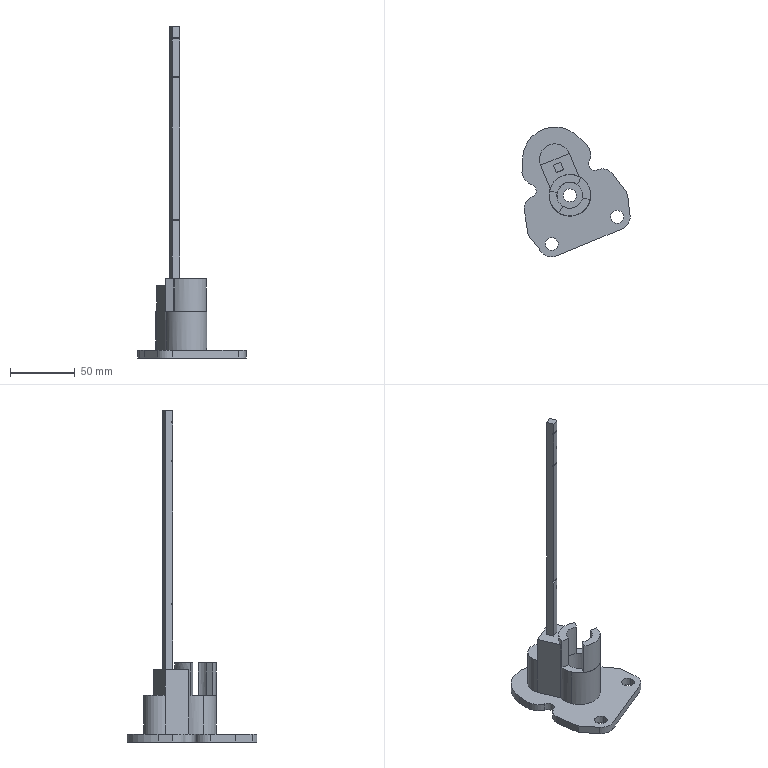Component | SolidWorks | MainFrame-1 | 1 solid | 69 faces | box 83.35 x 100.18 x 256 mm | volume 79027 mm3 | plane 41 | cylinder 26 | spline 2 | commonest cylinder face diameters 20 x10 10 x9 32 x3 20.1 x2 50 x1 24 x1
build123d program:
from build123d import *

# Parameters (mm, degrees)
SKETCH2_R             = 5
SKETCH2_R_2           = 10
BOSS_EXTRUDE1_DEPTH   = 6
SKETCH3_R             = 10
CUT_EXTRUDE1_DEPTH    = 3
SKETCH4_R             = 16
SKETCH4_R_2           = 10
BOSS_EXTRUDE2_DEPTH   = 30
BOSS_EXTRUDE3_DEPTH   = 50
BOSS_EXTRUDE4_DEPTH   = 25
SKETCH8_W             = 6
SKETCH8_H             = 6
BOSS_EXTRUDE5_DEPTH   = 200
CUT_EXTRUDE2_START    = -20
SKETCH10_R            = 10
CUT_EXTRUDE2_DEPTH    = 20
SKETCH11_W            = 1
SKETCH11_H            = 1
CUT_EXTRUDE3_DEPTH    = 10
SHAFTBORERELIEF_START = -30
SKETCH1_R             = 10.05
SHAFTBORERELIEF_DEPTH = 25


with BuildPart() as part:
    # Sketch2 → Boss-Extrude1 (new body)
    with BuildSketch(Plane.XY):
        with BuildLine():
            Line((-88.508, 57.757), (-33.948, 57.757))
            ThreePointArc((-33.948, 57.757), (-27.946, 55.756), (-24.347, 50.554))
            Line((-24.347, 50.554), (-19.716, 34.656))
            Line((-19.716, 34.656), (-24.233, 16.134))
            ThreePointArc((-24.233, 16.134), (-27.771, 10.639), (-33.948, 8.503))
            ThreePointArc((-33.948, 8.503), (-38.642, 5.225), (-37.182, -0.3102))
            add(Edge.make_bspline(
                [(-33.948, -12.168), (-32.916, -7.324), (-33.994, -3.371), (-37.182, -0.3102)],
                knots=[0, 0, 0, 0, 0.967, 0.967, 0.967, 0.967], degree=3))
            Line((-33.948, -12.168), (-38.577, -22.078))
            ThreePointArc((-38.577, -22.078), (-61.228, -36.497), (-83.878, -22.078))
            Line((-83.878, -22.078), (-88.508, -12.168))
            add(Edge.make_bspline(
                [(-88.508, -12.168), (-89.54, -7.324), (-88.462, -3.371), (-85.274, -0.3102)],
                knots=[0, 0, 0, 0, 0.967, 0.967, 0.967, 0.967], degree=3))
            ThreePointArc((-85.274, -0.3102), (-83.814, 5.225), (-88.508, 8.503))
            ThreePointArc((-88.508, 8.503), (-94.685, 10.639), (-98.223, 16.134))
            Line((-98.223, 16.134), (-102.739, 34.656))
            Line((-102.739, 34.656), (-98.109, 50.554))
            ThreePointArc((-98.109, 50.554), (-94.509, 55.756), (-88.508, 57.757))
        make_face()
        with Locations((-88.508, 47.757)):
            Circle(SKETCH2_R, mode=Mode.SUBTRACT)
        with Locations((-33.948, 47.757)):
            Circle(SKETCH2_R, mode=Mode.SUBTRACT)
        with Locations((-61.228, 18.503)):
            Circle(SKETCH2_R, mode=Mode.SUBTRACT)
        with Locations((-61.228, -11.497)):
            Circle(SKETCH2_R_2, mode=Mode.SUBTRACT)
    extrude(amount=BOSS_EXTRUDE1_DEPTH)

    # Sketch3 → Cut-Extrude1 (cut)
    with BuildSketch(Plane.XY.offset(6)):
        with Locations((-61.228, 18.503)):
            Circle(SKETCH3_R)
    extrude(amount=-CUT_EXTRUDE1_DEPTH, mode=Mode.SUBTRACT)

    # Sketch4 → Boss-Extrude2 (add)
    # profile 1 of 2: a face of its own
    with BuildSketch(Plane(origin=(0, 0, 0), x_dir=(-1, 0, 0), z_dir=(0, 0, -1))):
        with Locations(Location((61.228, 18.503, 0), (0, 0, 180))):
            Circle(SKETCH4_R)
        with Locations(Location((61.228, 18.503, 0), (0, 0, 180))):
            Circle(SKETCH4_R_2, mode=Mode.SUBTRACT)
    # profile 2 of 2: a face of its own
    with BuildSketch(Plane(origin=(0, 0, 0), x_dir=(-1, 0, 0), z_dir=(0, 0, -1))):
        with BuildLine():
            Line((73.228, -11.497), (71.228, -11.497))
            Line((71.228, -11.497), (51.228, -11.497))
            Line((51.228, -11.497), (49.228, -11.497))
            ThreePointArc((49.228, -11.497), (61.228, -23.497), (73.228, -11.497))
        make_face()
    extrude(amount=BOSS_EXTRUDE2_DEPTH)

    # Sketch5 → Boss-Extrude3 (add)
    with BuildSketch(Plane(origin=(0, 0, 0), x_dir=(-1, 0, 0), z_dir=(0, 0, -1))):
        with BuildLine():
            Line((49.228, -11.497), (49.228, 7.92))
            ThreePointArc((49.228, 7.92), (61.228, 2.503), (73.228, 7.92))
            Line((73.228, 7.92), (73.228, -11.497))
            Line((73.228, -11.497), (49.228, -11.497))
        make_face()
    extrude(amount=BOSS_EXTRUDE3_DEPTH)

    # Sketch6 → Boss-Extrude4 (add)
    with BuildSketch(Plane(origin=(0, 0, -30), x_dir=(-1, 0, 0), z_dir=(0, 0, -1))):
        with BuildLine():
            Line((48.079, 9.387), (53.01, 12.806))
            ThreePointArc((53.01, 12.806), (61.228, 8.503), (69.446, 12.806))
            Line((69.446, 12.806), (74.377, 9.387))
            ThreePointArc((74.377, 9.387), (73.824, 8.637), (73.228, 7.92))
            ThreePointArc((73.228, 7.92), (61.228, 2.503), (49.228, 7.92))
            ThreePointArc((49.228, 7.92), (48.632, 8.637), (48.079, 9.387))
        make_face()
    boss_extrude4 = extrude(amount=BOSS_EXTRUDE4_DEPTH)

    # Mirror1: Boss-Extrude4 across plane
    add(boss_extrude4.mirror(Plane.ZX.offset(18.5)))

    # Sketch8 → Boss-Extrude5 (add)
    with BuildSketch(Plane(origin=(0, 0, -50), x_dir=(-1, 0, 0), z_dir=(0, 0, -1))):
        with Locations((61.228, -4.497)):
            Rectangle(SKETCH8_W, SKETCH8_H)
    extrude(amount=BOSS_EXTRUDE5_DEPTH)

    # Sketch10 → Cut-Extrude2 (cut)
    with BuildSketch(Plane.XY.offset(CUT_EXTRUDE2_START)):
        with Locations((-61.228, -11.497)):
            Circle(SKETCH10_R)
    extrude(amount=CUT_EXTRUDE2_DEPTH, mode=Mode.SUBTRACT)

    # Sketch11 → Cut-Extrude3 (cut)
    with BuildSketch(Plane.ZY.offset(64.228)):
        with Locations((-240.5, -1.997)):
            Rectangle(SKETCH11_W, SKETCH11_H)
        with Locations((-100.5, -1.997)):
            Rectangle(SKETCH11_W, SKETCH11_H)
        with Locations((-210.5, -1.997)):
            Rectangle(SKETCH11_W, SKETCH11_H)
    extrude(amount=-CUT_EXTRUDE3_DEPTH, mode=Mode.SUBTRACT)

    # Sketch1 → ShaftBoreRelief (cut)
    with BuildSketch(Plane.XY.offset(SHAFTBORERELIEF_START)):
        with Locations((-61.228, 18.503)):
            Circle(SKETCH1_R)
    extrude(amount=-SHAFTBORERELIEF_DEPTH, mode=Mode.SUBTRACT)


solid = part.part

# Placed as in the assembly
solid = solid.moved(Location((78.431, 52.224, 142.846), (-180, 0, -22.523)))